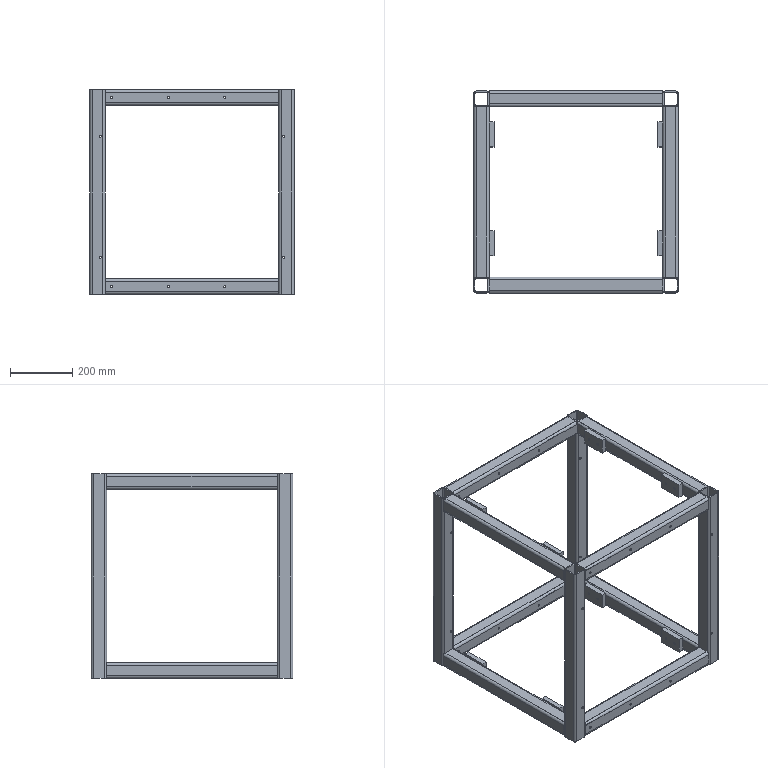Component | SolidWorks | JJ01-1 | 20 solids | 408 faces | volume 5414012 mm3 | cylinder 240 | plane 168 | commonest cylinder face diameters 7 x80 6.8 x64 16 x48 8 x48